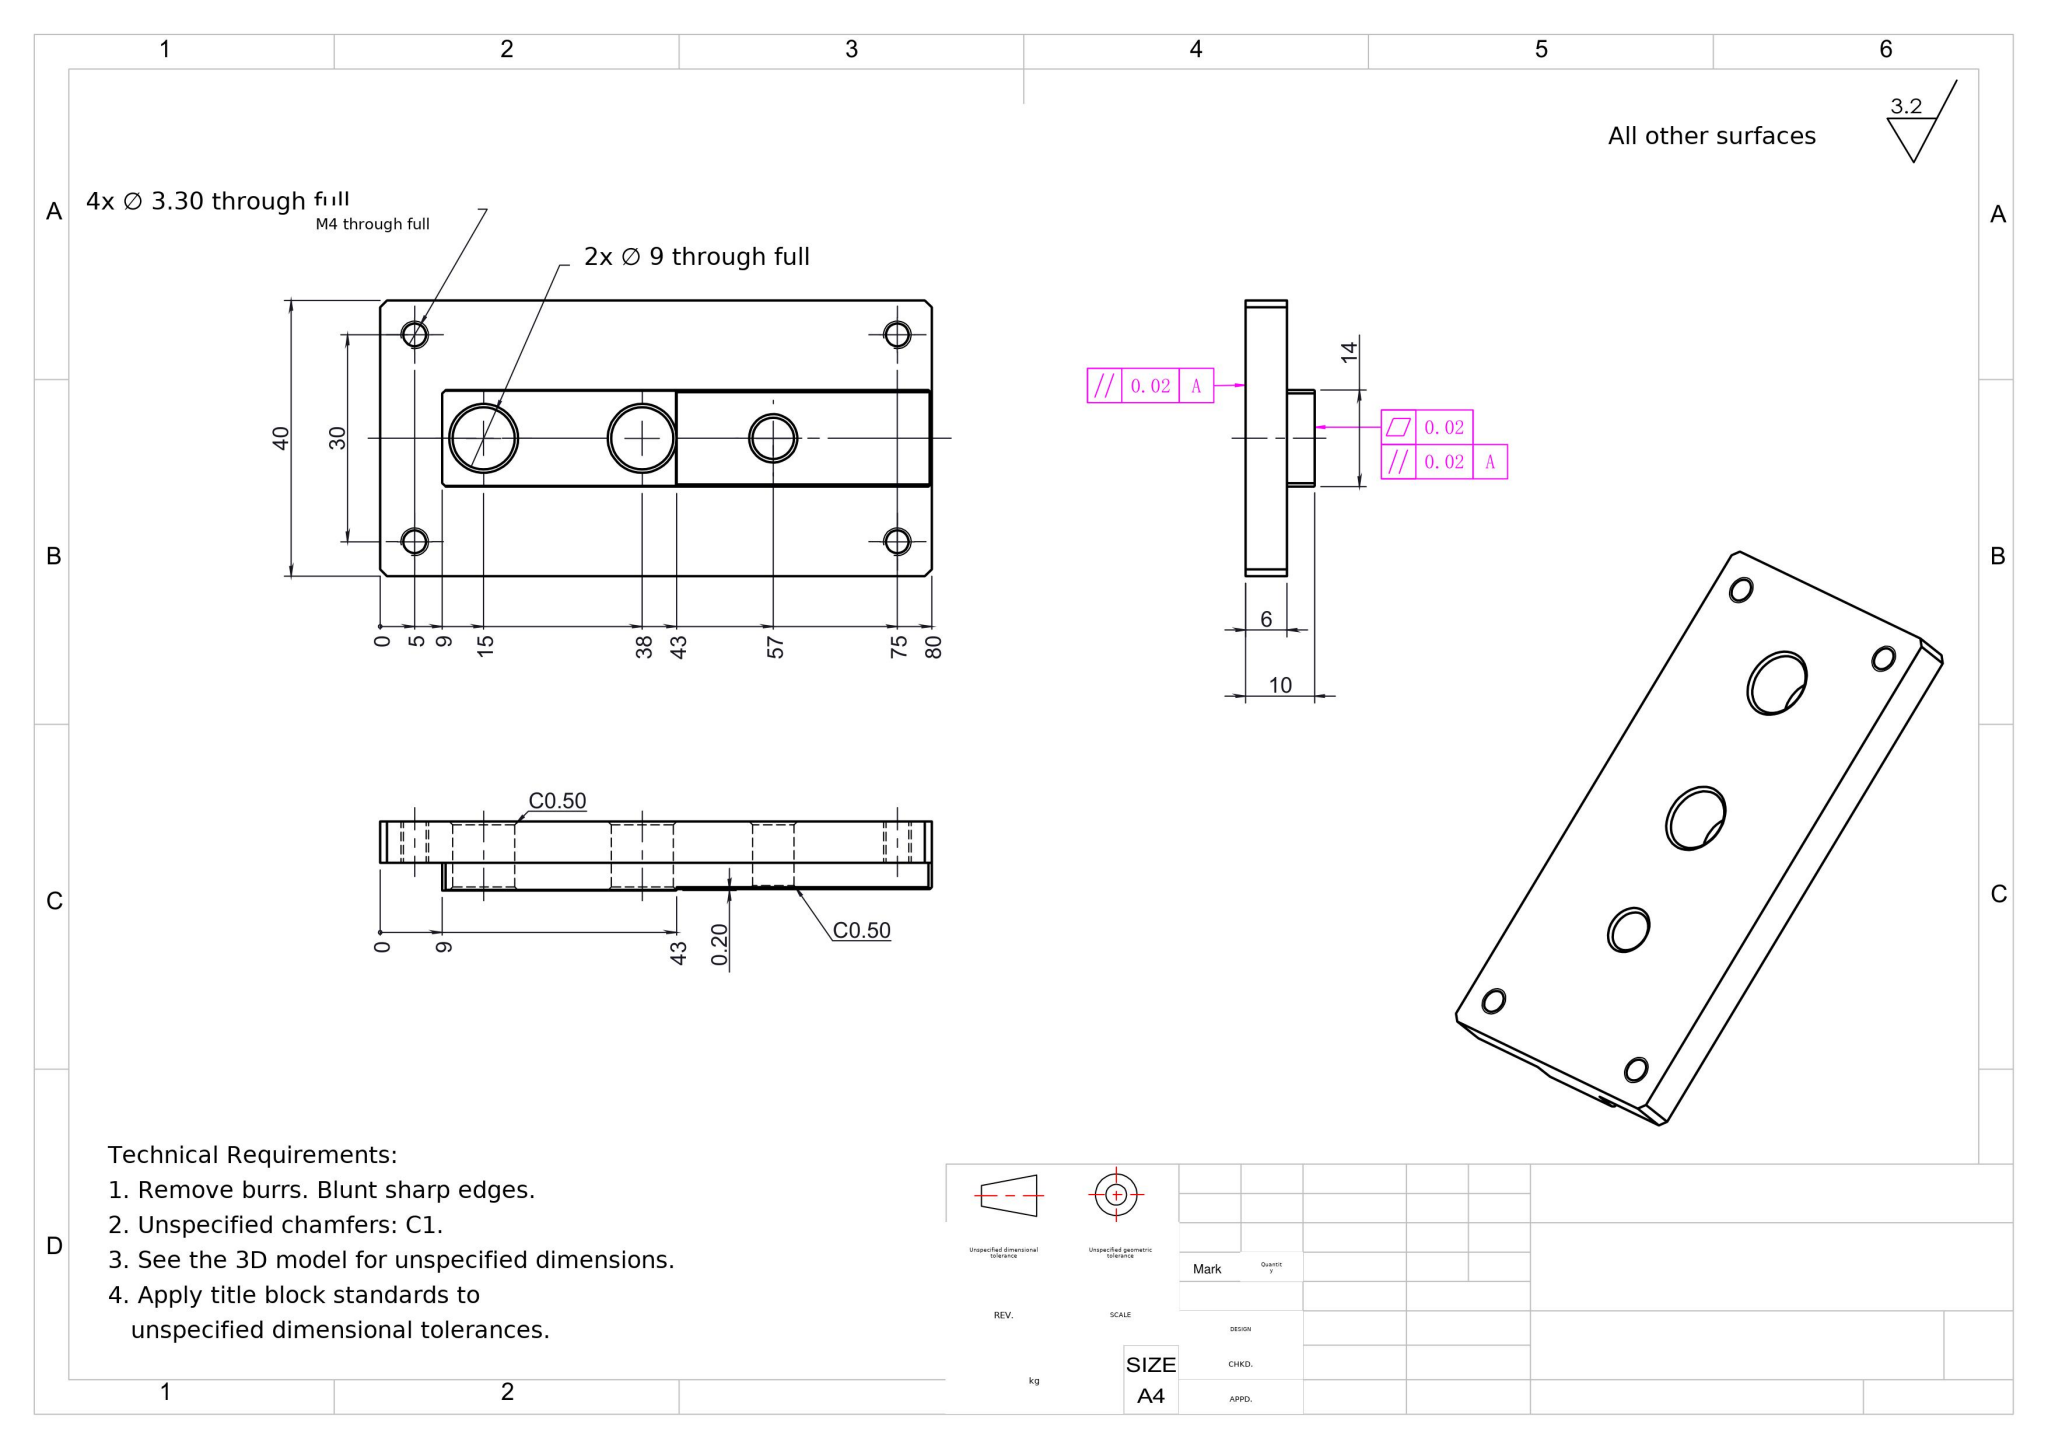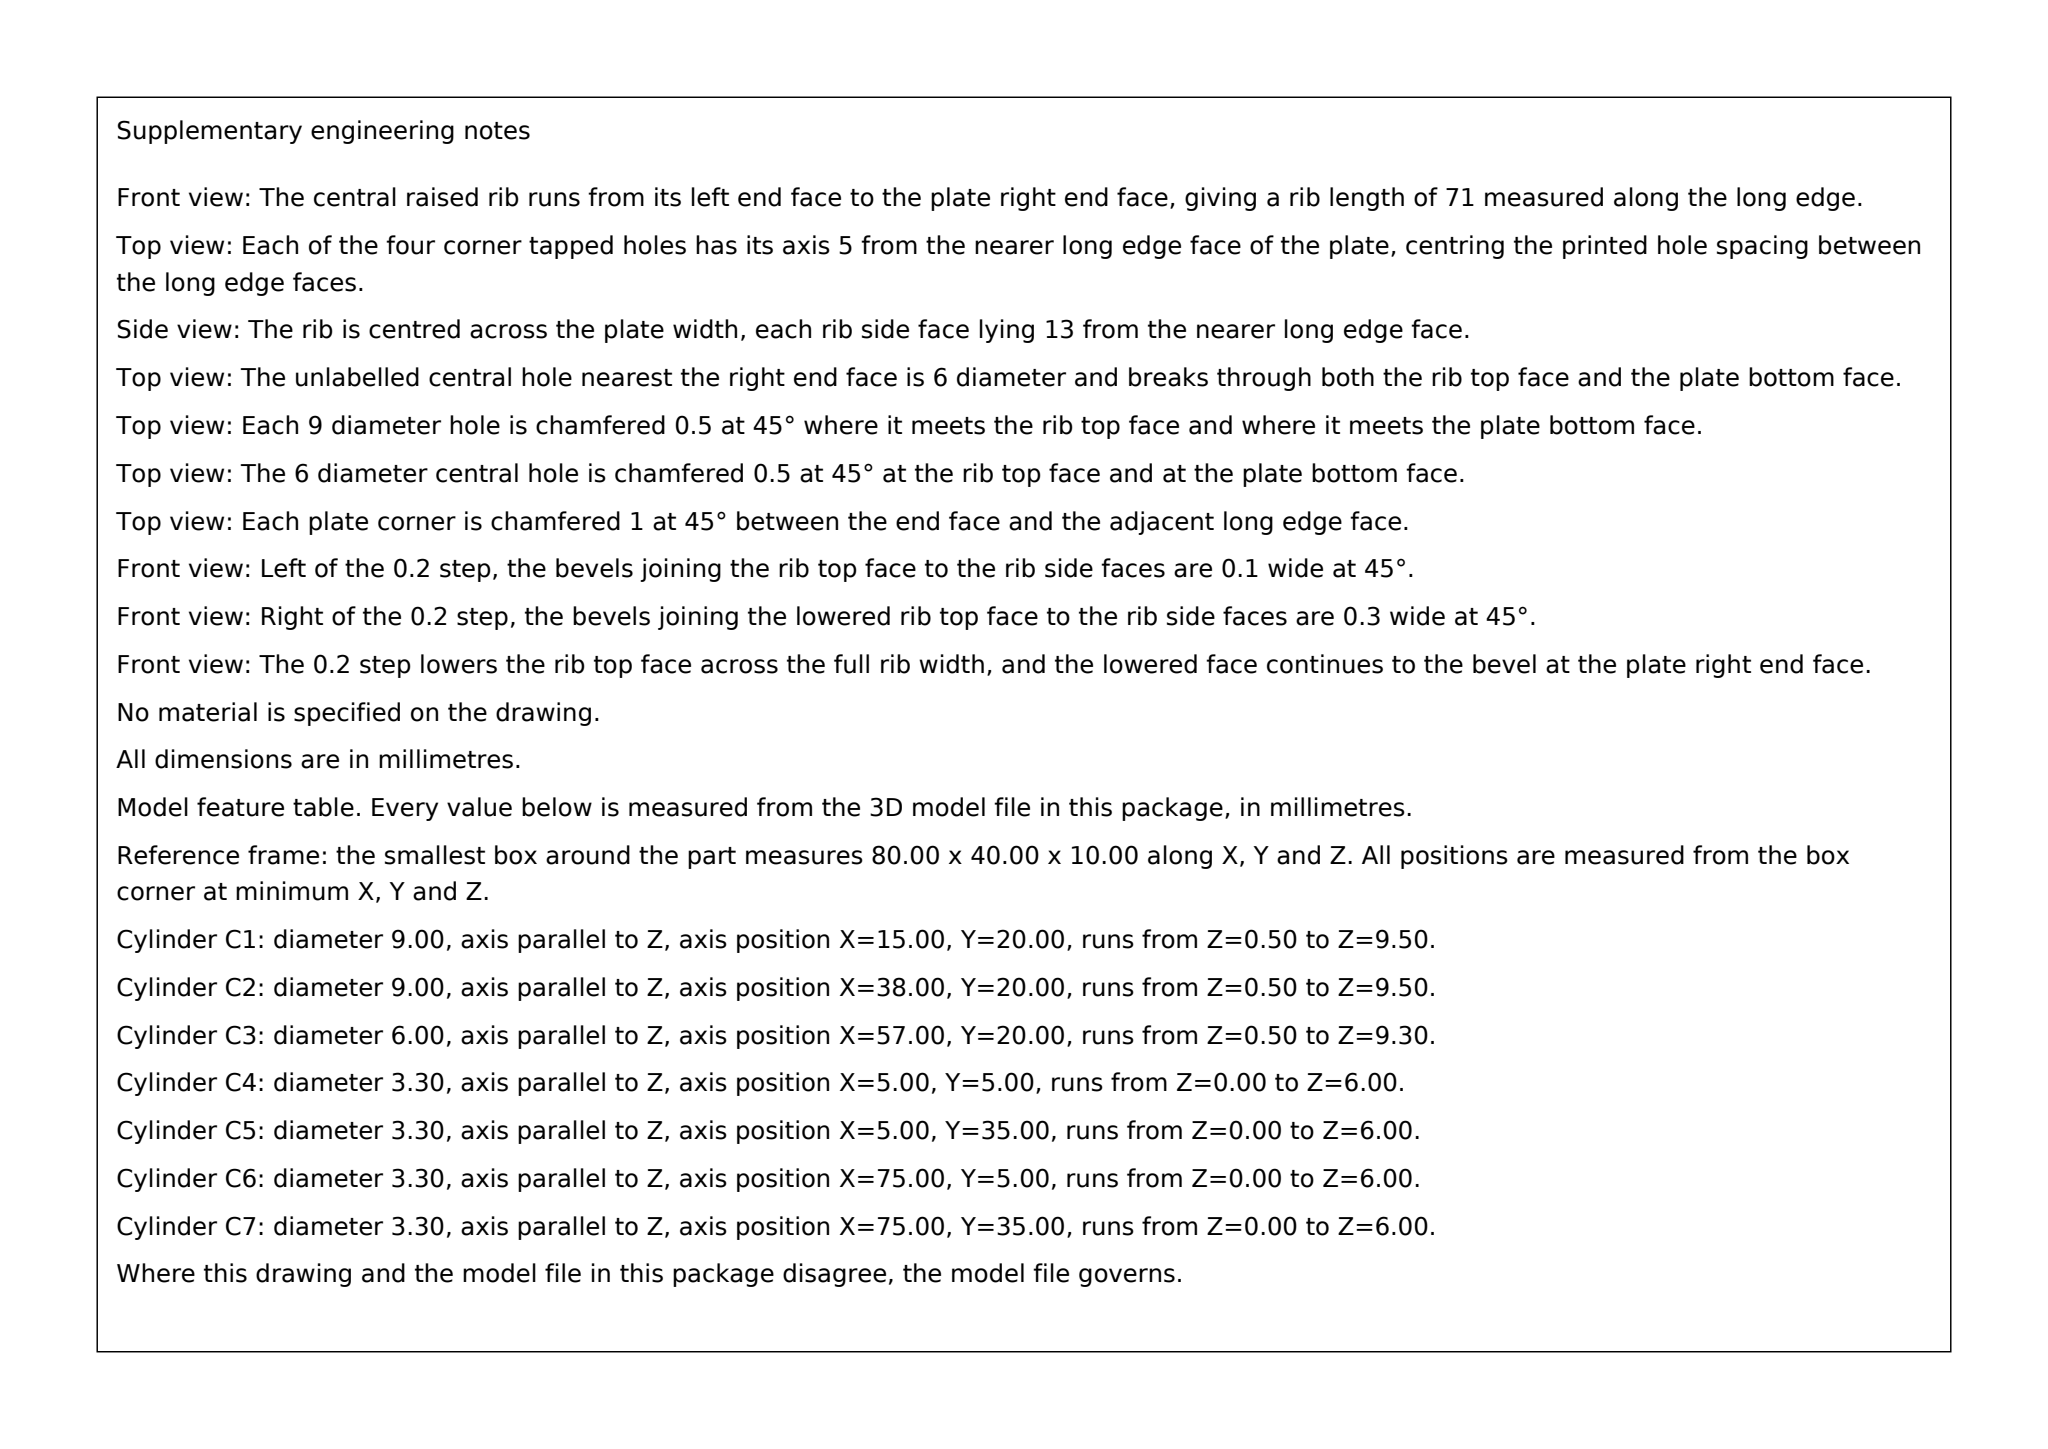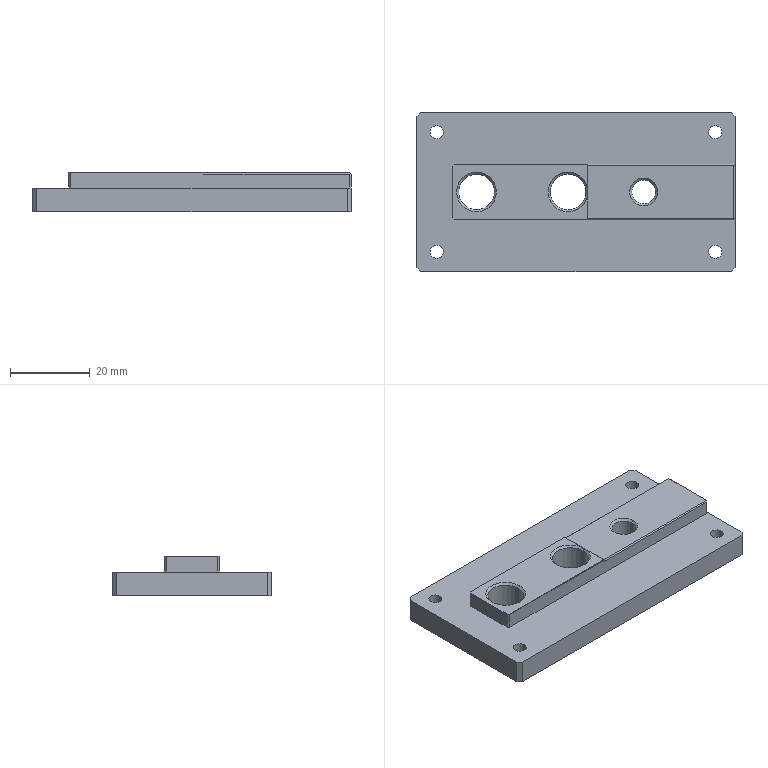Part | SolidWorks | mm | 1 solid | 52 faces | box 80 x 40 x 10 mm | volume 21280 mm3 | plane 26 | cylinder 14 | cone 12 | commonest cylinder face diameters 3.3 x8 9 x4 6 x2